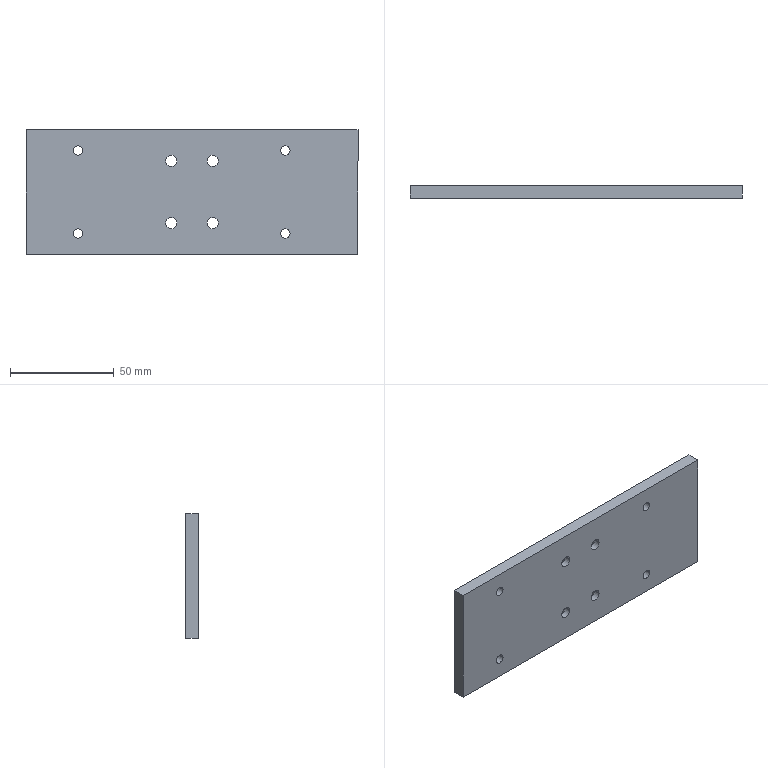Component | SolidWorks | CS021-A10-A007-1 | 1 solid | 30 faces | box 160 x 6 x 60 mm | volume 56270 mm3 | cylinder 16 | cone 8 | plane 6 | commonest cylinder face diameters 4.5 x8 5.5 x8 | material AL6061
build123d program:
from build123d import *

# Parameters (mm, degrees)
SKETCH1_W                                          = 160
SKETCH1_H                                          = 60
BOSS_EXTRUDE1_DEPTH                                = 3
HOLE_SIZE_ACCORDING_TO_SLOTTED_COUNTER_D           = 5.5
HOLE_SIZE_ACCORDING_TO_SLOTTED_COUNTER_CSINK_D     = 11.2
HOLE_SIZE_ACCORDING_TO_SLOTTED_COUNTER_CSINK_ANGLE = 90
F_4_5_4_5_DIAMETER_HOLE1_D                         = 4.5


with BuildPart() as part:
    # Sketch1 → Boss-Extrude1 (new, symmetric)
    with BuildSketch(Plane.XY):
        Rectangle(SKETCH1_W, SKETCH1_H)
    extrude(amount=BOSS_EXTRUDE1_DEPTH, both=True)

    # Hole Size _according to_ Slotted Counter (through all)
    with Locations(Plane.XY.offset(3)):
        with Locations((-10, 15), (10, 15), (10, -15), (-10, -15)):
            CounterSinkHole(HOLE_SIZE_ACCORDING_TO_SLOTTED_COUNTER_D / 2, HOLE_SIZE_ACCORDING_TO_SLOTTED_COUNTER_CSINK_D / 2, counter_sink_angle=HOLE_SIZE_ACCORDING_TO_SLOTTED_COUNTER_CSINK_ANGLE)

    # 4.5 _4.5_ Diameter Hole1 (through all)
    with Locations(Plane.XY.offset(3)):
        with Locations((-55.001, 20), (44.999, 20), (44.999, -20), (-55.001, -20)):
            Hole(F_4_5_4_5_DIAMETER_HOLE1_D / 2)


solid = part.part

# Placed as in the assembly
solid = solid.moved(Location((152.449, 155.317, 0), (-90, 0, 0)))
STEP:
#1=COLOUR_RGB('',0.7922,0.8196,0.9333);
#2=FILL_AREA_STYLE_COLOUR('',#1);
#3=FILL_AREA_STYLE('',(#2));
#4=SURFACE_STYLE_FILL_AREA(#3);
#5=SURFACE_SIDE_STYLE('',(#4));
#6=SURFACE_STYLE_USAGE(.BOTH.,#5);
#7=PRESENTATION_STYLE_ASSIGNMENT((#6));
#8=CARTESIAN_POINT('',(3.748,5.997,-0.7874));
#9=VERTEX_POINT('',#8);
#10=CARTESIAN_POINT('',(3.925,5.997,-0.7874));
#11=VERTEX_POINT('',#10);
#12=CARTESIAN_POINT('',(3.837,5.997,-0.7874));
#13=DIRECTION('',(-0.,1.,0.));
#14=DIRECTION('',(1.,0.,-0.));
#15=AXIS2_PLACEMENT_3D('',#12,#13,#14);
#16=CIRCLE('',#15,0.08858);
#17=EDGE_CURVE('',#9,#11,#16,.T.);
#18=ORIENTED_EDGE('',*,*,#17,.F.);
#19=CARTESIAN_POINT('',(3.748,6.233,-0.7874));
#20=VERTEX_POINT('',#19);
#21=CARTESIAN_POINT('',(3.748,6.233,-0.7874));
#22=DIRECTION('',(-0.,1.,0.));
#23=VECTOR('',#22,39.37);
#24=LINE('',#21,#23);
#25=EDGE_CURVE('',#9,#20,#24,.T.);
#26=ORIENTED_EDGE('',*,*,#25,.T.);
#27=CARTESIAN_POINT('',(3.925,6.233,-0.7874));
#28=VERTEX_POINT('',#27);
#29=CARTESIAN_POINT('',(3.837,6.233,-0.7874));
#30=DIRECTION('',(-0.,1.,0.));
#31=DIRECTION('',(1.,0.,-0.));
#32=AXIS2_PLACEMENT_3D('',#29,#30,#31);
#33=CIRCLE('',#32,0.08858);
#34=EDGE_CURVE('',#20,#28,#33,.T.);
#35=ORIENTED_EDGE('',*,*,#34,.T.);
#36=CARTESIAN_POINT('',(3.925,6.233,-0.7874));
#37=DIRECTION('',(-0.,1.,0.));
#38=VECTOR('',#37,39.37);
#39=LINE('',#36,#38);
#40=EDGE_CURVE('',#11,#28,#39,.T.);
#41=ORIENTED_EDGE('',*,*,#40,.F.);
#42=EDGE_LOOP('',(#18,#26,#35,#41));
#43=FACE_OUTER_BOUND('',#42,.T.);
#44=CARTESIAN_POINT('',(3.837,6.233,-0.7874));
#45=DIRECTION('',(-0.,1.,0.));
#46=DIRECTION('',(1.,0.,-0.));
#47=AXIS2_PLACEMENT_3D('',#44,#45,#46);
#48=CYLINDRICAL_SURFACE('',#47,0.08858);
#49=ADVANCED_FACE('',(#43),#48,.F.);
#50=CARTESIAN_POINT('',(7.685,5.997,-0.7874));
#51=VERTEX_POINT('',#50);
#52=CARTESIAN_POINT('',(7.862,5.997,-0.7874));
#53=VERTEX_POINT('',#52);
#54=CARTESIAN_POINT('',(7.774,5.997,-0.7874));
#55=DIRECTION('',(-0.,1.,0.));
#56=DIRECTION('',(1.,0.,-0.));
#57=AXIS2_PLACEMENT_3D('',#54,#55,#56);
#58=CIRCLE('',#57,0.08858);
#59=EDGE_CURVE('',#51,#53,#58,.T.);
#60=ORIENTED_EDGE('',*,*,#59,.F.);
#61=CARTESIAN_POINT('',(7.685,6.233,-0.7874));
#62=VERTEX_POINT('',#61);
#63=CARTESIAN_POINT('',(7.685,6.233,-0.7874));
#64=DIRECTION('',(-0.,1.,0.));
#65=VECTOR('',#64,39.37);
#66=LINE('',#63,#65);
#67=EDGE_CURVE('',#51,#62,#66,.T.);
#68=ORIENTED_EDGE('',*,*,#67,.T.);
#69=CARTESIAN_POINT('',(7.862,6.233,-0.7874));
#70=VERTEX_POINT('',#69);
#71=CARTESIAN_POINT('',(7.774,6.233,-0.7874));
#72=DIRECTION('',(-0.,1.,0.));
#73=DIRECTION('',(1.,0.,-0.));
#74=AXIS2_PLACEMENT_3D('',#71,#72,#73);
#75=CIRCLE('',#74,0.08858);
#76=EDGE_CURVE('',#62,#70,#75,.T.);
#77=ORIENTED_EDGE('',*,*,#76,.T.);
#78=CARTESIAN_POINT('',(7.862,6.233,-0.7874));
#79=DIRECTION('',(-0.,1.,0.));
#80=VECTOR('',#79,39.37);
#81=LINE('',#78,#80);
#82=EDGE_CURVE('',#53,#70,#81,.T.);
#83=ORIENTED_EDGE('',*,*,#82,.F.);
#84=EDGE_LOOP('',(#60,#68,#77,#83));
#85=FACE_OUTER_BOUND('',#84,.T.);
#86=CARTESIAN_POINT('',(7.774,6.233,-0.7874));
#87=DIRECTION('',(-0.,1.,0.));
#88=DIRECTION('',(1.,0.,-0.));
#89=AXIS2_PLACEMENT_3D('',#86,#87,#88);
#90=CYLINDRICAL_SURFACE('',#89,0.08858);
#91=ADVANCED_FACE('',(#85),#90,.F.);
#92=CARTESIAN_POINT('',(7.685,5.997,0.7874));
#93=VERTEX_POINT('',#92);
#94=CARTESIAN_POINT('',(7.862,5.997,0.7874));
#95=VERTEX_POINT('',#94);
#96=CARTESIAN_POINT('',(7.774,5.997,0.7874));
#97=DIRECTION('',(-0.,1.,0.));
#98=DIRECTION('',(1.,0.,-0.));
#99=AXIS2_PLACEMENT_3D('',#96,#97,#98);
#100=CIRCLE('',#99,0.08858);
#101=EDGE_CURVE('',#93,#95,#100,.T.);
#102=ORIENTED_EDGE('',*,*,#101,.F.);
#103=CARTESIAN_POINT('',(7.685,6.233,0.7874));
#104=VERTEX_POINT('',#103);
#105=CARTESIAN_POINT('',(7.685,6.233,0.7874));
#106=DIRECTION('',(-0.,1.,0.));
#107=VECTOR('',#106,39.37);
#108=LINE('',#105,#107);
#109=EDGE_CURVE('',#93,#104,#108,.T.);
#110=ORIENTED_EDGE('',*,*,#109,.T.);
#111=CARTESIAN_POINT('',(7.862,6.233,0.7874));
#112=VERTEX_POINT('',#111);
#113=CARTESIAN_POINT('',(7.774,6.233,0.7874));
#114=DIRECTION('',(-0.,1.,0.));
#115=DIRECTION('',(1.,0.,-0.));
#116=AXIS2_PLACEMENT_3D('',#113,#114,#115);
#117=CIRCLE('',#116,0.08858);
#118=EDGE_CURVE('',#104,#112,#117,.T.);
#119=ORIENTED_EDGE('',*,*,#118,.T.);
#120=CARTESIAN_POINT('',(7.862,6.233,0.7874));
#121=DIRECTION('',(-0.,1.,0.));
#122=VECTOR('',#121,39.37);
#123=LINE('',#120,#122);
#124=EDGE_CURVE('',#95,#112,#123,.T.);
#125=ORIENTED_EDGE('',*,*,#124,.F.);
#126=EDGE_LOOP('',(#102,#110,#119,#125));
#127=FACE_OUTER_BOUND('',#126,.T.);
#128=CARTESIAN_POINT('',(7.774,6.233,0.7874));
#129=DIRECTION('',(-0.,1.,0.));
#130=DIRECTION('',(1.,0.,-0.));
#131=AXIS2_PLACEMENT_3D('',#128,#129,#130);
#132=CYLINDRICAL_SURFACE('',#131,0.08858);
#133=ADVANCED_FACE('',(#127),#132,.F.);
#134=CARTESIAN_POINT('',(3.748,5.997,0.7874));
#135=VERTEX_POINT('',#134);
#136=CARTESIAN_POINT('',(3.925,5.997,0.7874));
#137=VERTEX_POINT('',#136);
#138=CARTESIAN_POINT('',(3.837,5.997,0.7874));
#139=DIRECTION('',(-0.,1.,0.));
#140=DIRECTION('',(1.,0.,-0.));
#141=AXIS2_PLACEMENT_3D('',#138,#139,#140);
#142=CIRCLE('',#141,0.08858);
#143=EDGE_CURVE('',#135,#137,#142,.T.);
#144=ORIENTED_EDGE('',*,*,#143,.F.);
#145=CARTESIAN_POINT('',(3.748,6.233,0.7874));
#146=VERTEX_POINT('',#145);
#147=CARTESIAN_POINT('',(3.748,6.233,0.7874));
#148=DIRECTION('',(-0.,1.,0.));
#149=VECTOR('',#148,39.37);
#150=LINE('',#147,#149);
#151=EDGE_CURVE('',#135,#146,#150,.T.);
#152=ORIENTED_EDGE('',*,*,#151,.T.);
#153=CARTESIAN_POINT('',(3.925,6.233,0.7874));
#154=VERTEX_POINT('',#153);
#155=CARTESIAN_POINT('',(3.837,6.233,0.7874));
#156=DIRECTION('',(-0.,1.,0.));
#157=DIRECTION('',(1.,0.,-0.));
#158=AXIS2_PLACEMENT_3D('',#155,#156,#157);
#159=CIRCLE('',#158,0.08858);
#160=EDGE_CURVE('',#146,#154,#159,.T.);
#161=ORIENTED_EDGE('',*,*,#160,.T.);
#162=CARTESIAN_POINT('',(3.925,6.233,0.7874));
#163=DIRECTION('',(-0.,1.,0.));
#164=VECTOR('',#163,39.37);
#165=LINE('',#162,#164);
#166=EDGE_CURVE('',#137,#154,#165,.T.);
#167=ORIENTED_EDGE('',*,*,#166,.F.);
#168=EDGE_LOOP('',(#144,#152,#161,#167));
#169=FACE_OUTER_BOUND('',#168,.T.);
#170=CARTESIAN_POINT('',(3.837,6.233,0.7874));
#171=DIRECTION('',(-0.,1.,0.));
#172=DIRECTION('',(1.,0.,-0.));
#173=AXIS2_PLACEMENT_3D('',#170,#171,#172);
#174=CYLINDRICAL_SURFACE('',#173,0.08858);
#175=ADVANCED_FACE('',(#169),#174,.F.);
#176=CARTESIAN_POINT('',(5.5,6.121,-0.5906));
#177=VERTEX_POINT('',#176);
#178=CARTESIAN_POINT('',(5.716,6.121,-0.5906));
#179=VERTEX_POINT('',#178);
#180=CARTESIAN_POINT('',(5.608,6.121,-0.5906));
#181=DIRECTION('',(-0.,1.,0.));
#182=DIRECTION('',(1.,0.,-0.));
#183=AXIS2_PLACEMENT_3D('',#180,#181,#182);
#184=CIRCLE('',#183,0.1083);
#185=EDGE_CURVE('',#177,#179,#184,.T.);
#186=ORIENTED_EDGE('',*,*,#185,.F.);
#187=CARTESIAN_POINT('',(5.388,6.233,-0.5906));
#188=VERTEX_POINT('',#187);
#189=CARTESIAN_POINT('',(5.388,6.233,-0.5906));
#190=DIRECTION('',(-0.7071,0.7071,0.));
#191=VECTOR('',#190,39.37);
#192=LINE('',#189,#191);
#193=EDGE_CURVE('',#177,#188,#192,.T.);
#194=ORIENTED_EDGE('',*,*,#193,.T.);
#195=CARTESIAN_POINT('',(5.829,6.233,-0.5906));
#196=VERTEX_POINT('',#195);
#197=CARTESIAN_POINT('',(5.608,6.233,-0.5906));
#198=DIRECTION('',(-0.,1.,0.));
#199=DIRECTION('',(1.,0.,-0.));
#200=AXIS2_PLACEMENT_3D('',#197,#198,#199);
#201=CIRCLE('',#200,0.2205);
#202=EDGE_CURVE('',#188,#196,#201,.T.);
#203=ORIENTED_EDGE('',*,*,#202,.T.);
#204=CARTESIAN_POINT('',(5.829,6.233,-0.5906));
#205=DIRECTION('',(0.7071,0.7071,-0.));
#206=VECTOR('',#205,39.37);
#207=LINE('',#204,#206);
#208=EDGE_CURVE('',#179,#196,#207,.T.);
#209=ORIENTED_EDGE('',*,*,#208,.F.);
#210=EDGE_LOOP('',(#186,#194,#203,#209));
#211=FACE_OUTER_BOUND('',#210,.T.);
#212=CARTESIAN_POINT('',(5.608,6.233,-0.5906));
#213=DIRECTION('',(-0.,1.,0.));
#214=DIRECTION('',(1.,0.,-0.));
#215=AXIS2_PLACEMENT_3D('',#212,#213,#214);
#216=CONICAL_SURFACE('',#215,0.2205,0.7854);
#217=ADVANCED_FACE('',(#211),#216,.F.);
#218=CARTESIAN_POINT('',(5.5,5.997,-0.5906));
#219=VERTEX_POINT('',#218);
#220=CARTESIAN_POINT('',(5.716,5.997,-0.5906));
#221=VERTEX_POINT('',#220);
#222=CARTESIAN_POINT('',(5.608,5.997,-0.5906));
#223=DIRECTION('',(-0.,1.,0.));
#224=DIRECTION('',(1.,0.,-0.));
#225=AXIS2_PLACEMENT_3D('',#222,#223,#224);
#226=CIRCLE('',#225,0.1083);
#227=EDGE_CURVE('',#219,#221,#226,.T.);
#228=ORIENTED_EDGE('',*,*,#227,.F.);
#229=CARTESIAN_POINT('',(5.5,6.233,-0.5906));
#230=DIRECTION('',(-0.,1.,0.));
#231=VECTOR('',#230,39.37);
#232=LINE('',#229,#231);
#233=EDGE_CURVE('',#219,#177,#232,.T.);
#234=ORIENTED_EDGE('',*,*,#233,.T.);
#235=ORIENTED_EDGE('',*,*,#185,.T.);
#236=CARTESIAN_POINT('',(5.716,6.233,-0.5906));
#237=DIRECTION('',(-0.,1.,0.));
#238=VECTOR('',#237,39.37);
#239=LINE('',#236,#238);
#240=EDGE_CURVE('',#221,#179,#239,.T.);
#241=ORIENTED_EDGE('',*,*,#240,.F.);
#242=EDGE_LOOP('',(#228,#234,#235,#241));
#243=FACE_OUTER_BOUND('',#242,.T.);
#244=CARTESIAN_POINT('',(5.608,6.233,-0.5906));
#245=DIRECTION('',(-0.,1.,0.));
#246=DIRECTION('',(1.,0.,-0.));
#247=AXIS2_PLACEMENT_3D('',#244,#245,#246);
#248=CYLINDRICAL_SURFACE('',#247,0.1083);
#249=ADVANCED_FACE('',(#243),#248,.F.);
#250=CARTESIAN_POINT('',(6.287,6.121,-0.5906));
#251=VERTEX_POINT('',#250);
#252=CARTESIAN_POINT('',(6.504,6.121,-0.5906));
#253=VERTEX_POINT('',#252);
#254=CARTESIAN_POINT('',(6.396,6.121,-0.5906));
#255=DIRECTION('',(-0.,1.,0.));
#256=DIRECTION('',(1.,0.,-0.));
#257=AXIS2_PLACEMENT_3D('',#254,#255,#256);
#258=CIRCLE('',#257,0.1083);
#259=EDGE_CURVE('',#251,#253,#258,.T.);
#260=ORIENTED_EDGE('',*,*,#259,.F.);
#261=CARTESIAN_POINT('',(6.175,6.233,-0.5906));
#262=VERTEX_POINT('',#261);
#263=CARTESIAN_POINT('',(6.175,6.233,-0.5906));
#264=DIRECTION('',(-0.7071,0.7071,0.));
#265=VECTOR('',#264,39.37);
#266=LINE('',#263,#265);
#267=EDGE_CURVE('',#251,#262,#266,.T.);
#268=ORIENTED_EDGE('',*,*,#267,.T.);
#269=CARTESIAN_POINT('',(6.616,6.233,-0.5906));
#270=VERTEX_POINT('',#269);
#271=CARTESIAN_POINT('',(6.396,6.233,-0.5906));
#272=DIRECTION('',(-0.,1.,0.));
#273=DIRECTION('',(1.,0.,-0.));
#274=AXIS2_PLACEMENT_3D('',#271,#272,#273);
#275=CIRCLE('',#274,0.2205);
#276=EDGE_CURVE('',#262,#270,#275,.T.);
#277=ORIENTED_EDGE('',*,*,#276,.T.);
#278=CARTESIAN_POINT('',(6.616,6.233,-0.5906));
#279=DIRECTION('',(0.7071,0.7071,-0.));
#280=VECTOR('',#279,39.37);
#281=LINE('',#278,#280);
#282=EDGE_CURVE('',#253,#270,#281,.T.);
#283=ORIENTED_EDGE('',*,*,#282,.F.);
#284=EDGE_LOOP('',(#260,#268,#277,#283));
#285=FACE_OUTER_BOUND('',#284,.T.);
#286=CARTESIAN_POINT('',(6.396,6.233,-0.5906));
#287=DIRECTION('',(-0.,1.,0.));
#288=DIRECTION('',(1.,0.,-0.));
#289=AXIS2_PLACEMENT_3D('',#286,#287,#288);
#290=CONICAL_SURFACE('',#289,0.2205,0.7854);
#291=ADVANCED_FACE('',(#285),#290,.F.);
#292=CARTESIAN_POINT('',(6.287,5.997,-0.5906));
#293=VERTEX_POINT('',#292);
#294=CARTESIAN_POINT('',(6.504,5.997,-0.5906));
#295=VERTEX_POINT('',#294);
#296=CARTESIAN_POINT('',(6.396,5.997,-0.5906));
#297=DIRECTION('',(-0.,1.,0.));
#298=DIRECTION('',(1.,0.,-0.));
#299=AXIS2_PLACEMENT_3D('',#296,#297,#298);
#300=CIRCLE('',#299,0.1083);
#301=EDGE_CURVE('',#293,#295,#300,.T.);
#302=ORIENTED_EDGE('',*,*,#301,.F.);
#303=CARTESIAN_POINT('',(6.287,6.233,-0.5906));
#304=DIRECTION('',(-0.,1.,0.));
#305=VECTOR('',#304,39.37);
#306=LINE('',#303,#305);
#307=EDGE_CURVE('',#293,#251,#306,.T.);
#308=ORIENTED_EDGE('',*,*,#307,.T.);
#309=ORIENTED_EDGE('',*,*,#259,.T.);
#310=CARTESIAN_POINT('',(6.504,6.233,-0.5906));
#311=DIRECTION('',(-0.,1.,0.));
#312=VECTOR('',#311,39.37);
#313=LINE('',#310,#312);
#314=EDGE_CURVE('',#295,#253,#313,.T.);
#315=ORIENTED_EDGE('',*,*,#314,.F.);
#316=EDGE_LOOP('',(#302,#308,#309,#315));
#317=FACE_OUTER_BOUND('',#316,.T.);
#318=CARTESIAN_POINT('',(6.396,6.233,-0.5906));
#319=DIRECTION('',(-0.,1.,0.));
#320=DIRECTION('',(1.,0.,-0.));
#321=AXIS2_PLACEMENT_3D('',#318,#319,#320);
#322=CYLINDRICAL_SURFACE('',#321,0.1083);
#323=ADVANCED_FACE('',(#317),#322,.F.);
#324=CARTESIAN_POINT('',(6.287,6.121,0.5906));
#325=VERTEX_POINT('',#324);
#326=CARTESIAN_POINT('',(6.504,6.121,0.5906));
#327=VERTEX_POINT('',#326);
#328=CARTESIAN_POINT('',(6.396,6.121,0.5906));
#329=DIRECTION('',(-0.,1.,0.));
#330=DIRECTION('',(1.,0.,-0.));
#331=AXIS2_PLACEMENT_3D('',#328,#329,#330);
#332=CIRCLE('',#331,0.1083);
#333=EDGE_CURVE('',#325,#327,#332,.T.);
#334=ORIENTED_EDGE('',*,*,#333,.F.);
#335=CARTESIAN_POINT('',(6.175,6.233,0.5906));
#336=VERTEX_POINT('',#335);
#337=CARTESIAN_POINT('',(6.175,6.233,0.5906));
#338=DIRECTION('',(-0.7071,0.7071,0.));
#339=VECTOR('',#338,39.37);
#340=LINE('',#337,#339);
#341=EDGE_CURVE('',#325,#336,#340,.T.);
#342=ORIENTED_EDGE('',*,*,#341,.T.);
#343=CARTESIAN_POINT('',(6.616,6.233,0.5906));
#344=VERTEX_POINT('',#343);
#345=CARTESIAN_POINT('',(6.396,6.233,0.5906));
#346=DIRECTION('',(-0.,1.,0.));
#347=DIRECTION('',(1.,0.,-0.));
#348=AXIS2_PLACEMENT_3D('',#345,#346,#347);
#349=CIRCLE('',#348,0.2205);
#350=EDGE_CURVE('',#336,#344,#349,.T.);
#351=ORIENTED_EDGE('',*,*,#350,.T.);
#352=CARTESIAN_POINT('',(6.616,6.233,0.5906));
#353=DIRECTION('',(0.7071,0.7071,-0.));
#354=VECTOR('',#353,39.37);
#355=LINE('',#352,#354);
#356=EDGE_CURVE('',#327,#344,#355,.T.);
#357=ORIENTED_EDGE('',*,*,#356,.F.);
#358=EDGE_LOOP('',(#334,#342,#351,#357));
#359=FACE_OUTER_BOUND('',#358,.T.);
#360=CARTESIAN_POINT('',(6.396,6.233,0.5906));
#361=DIRECTION('',(-0.,1.,0.));
#362=DIRECTION('',(1.,0.,-0.));
#363=AXIS2_PLACEMENT_3D('',#360,#361,#362);
#364=CONICAL_SURFACE('',#363,0.2205,0.7854);
#365=ADVANCED_FACE('',(#359),#364,.F.);
#366=CARTESIAN_POINT('',(6.287,5.997,0.5906));
#367=VERTEX_POINT('',#366);
#368=CARTESIAN_POINT('',(6.504,5.997,0.5906));
#369=VERTEX_POINT('',#368);
#370=CARTESIAN_POINT('',(6.396,5.997,0.5906));
#371=DIRECTION('',(-0.,1.,0.));
#372=DIRECTION('',(1.,0.,-0.));
#373=AXIS2_PLACEMENT_3D('',#370,#371,#372);
#374=CIRCLE('',#373,0.1083);
#375=EDGE_CURVE('',#367,#369,#374,.T.);
#376=ORIENTED_EDGE('',*,*,#375,.F.);
#377=CARTESIAN_POINT('',(6.287,6.233,0.5906));
#378=DIRECTION('',(-0.,1.,0.));
#379=VECTOR('',#378,39.37);
#380=LINE('',#377,#379);
#381=EDGE_CURVE('',#367,#325,#380,.T.);
#382=ORIENTED_EDGE('',*,*,#381,.T.);
#383=ORIENTED_EDGE('',*,*,#333,.T.);
#384=CARTESIAN_POINT('',(6.504,6.233,0.5906));
#385=DIRECTION('',(-0.,1.,0.));
#386=VECTOR('',#385,39.37);
#387=LINE('',#384,#386);
#388=EDGE_CURVE('',#369,#327,#387,.T.);
#389=ORIENTED_EDGE('',*,*,#388,.F.);
#390=EDGE_LOOP('',(#376,#382,#383,#389));
#391=FACE_OUTER_BOUND('',#390,.T.);
#392=CARTESIAN_POINT('',(6.396,6.233,0.5906));
#393=DIRECTION('',(-0.,1.,0.));
#394=DIRECTION('',(1.,0.,-0.));
#395=AXIS2_PLACEMENT_3D('',#392,#393,#394);
#396=CYLINDRICAL_SURFACE('',#395,0.1083);
#397=ADVANCED_FACE('',(#391),#396,.F.);
#398=CARTESIAN_POINT('',(5.5,6.121,0.5906));
#399=VERTEX_POINT('',#398);
#400=CARTESIAN_POINT('',(5.716,6.121,0.5906));
#401=VERTEX_POINT('',#400);
#402=CARTESIAN_POINT('',(5.608,6.121,0.5906));
#403=DIRECTION('',(-0.,1.,0.));
#404=DIRECTION('',(1.,0.,-0.));
#405=AXIS2_PLACEMENT_3D('',#402,#403,#404);
#406=CIRCLE('',#405,0.1083);
#407=EDGE_CURVE('',#399,#401,#406,.T.);
#408=ORIENTED_EDGE('',*,*,#407,.F.);
#409=CARTESIAN_POINT('',(5.388,6.233,0.5906));
#410=VERTEX_POINT('',#409);
#411=CARTESIAN_POINT('',(5.388,6.233,0.5906));
#412=DIRECTION('',(-0.7071,0.7071,0.));
#413=VECTOR('',#412,39.37);
#414=LINE('',#411,#413);
#415=EDGE_CURVE('',#399,#410,#414,.T.);
#416=ORIENTED_EDGE('',*,*,#415,.T.);
#417=CARTESIAN_POINT('',(5.829,6.233,0.5906));
#418=VERTEX_POINT('',#417);
#419=CARTESIAN_POINT('',(5.608,6.233,0.5906));
#420=DIRECTION('',(-0.,1.,0.));
#421=DIRECTION('',(1.,0.,-0.));
#422=AXIS2_PLACEMENT_3D('',#419,#420,#421);
#423=CIRCLE('',#422,0.2205);
#424=EDGE_CURVE('',#410,#418,#423,.T.);
#425=ORIENTED_EDGE('',*,*,#424,.T.);
#426=CARTESIAN_POINT('',(5.829,6.233,0.5906));
#427=DIRECTION('',(0.7071,0.7071,-0.));
#428=VECTOR('',#427,39.37);
#429=LINE('',#426,#428);
#430=EDGE_CURVE('',#401,#418,#429,.T.);
#431=ORIENTED_EDGE('',*,*,#430,.F.);
#432=EDGE_LOOP('',(#408,#416,#425,#431));
#433=FACE_OUTER_BOUND('',#432,.T.);
#434=CARTESIAN_POINT('',(5.608,6.233,0.5906));
#435=DIRECTION('',(-0.,1.,0.));
#436=DIRECTION('',(1.,0.,-0.));
#437=AXIS2_PLACEMENT_3D('',#434,#435,#436);
#438=CONICAL_SURFACE('',#437,0.2205,0.7854);
#439=ADVANCED_FACE('',(#433),#438,.F.);
#440=CARTESIAN_POINT('',(5.5,5.997,0.5906));
#441=VERTEX_POINT('',#440);
#442=CARTESIAN_POINT('',(5.716,5.997,0.5906));
#443=VERTEX_POINT('',#442);
#444=CARTESIAN_POINT('',(5.608,5.997,0.5906));
#445=DIRECTION('',(-0.,1.,0.));
#446=DIRECTION('',(1.,0.,-0.));
#447=AXIS2_PLACEMENT_3D('',#444,#445,#446);
#448=CIRCLE('',#447,0.1083);
#449=EDGE_CURVE('',#441,#443,#448,.T.);
#450=ORIENTED_EDGE('',*,*,#449,.F.);
#451=CARTESIAN_POINT('',(5.5,6.233,0.5906));
#452=DIRECTION('',(-0.,1.,0.));
#453=VECTOR('',#452,39.37);
#454=LINE('',#451,#453);
#455=EDGE_CURVE('',#441,#399,#454,.T.);
#456=ORIENTED_EDGE('',*,*,#455,.T.);
#457=ORIENTED_EDGE('',*,*,#407,.T.);
#458=CARTESIAN_POINT('',(5.716,6.233,0.5906));
#459=DIRECTION('',(-0.,1.,0.));
#460=VECTOR('',#459,39.37);
#461=LINE('',#458,#460);
#462=EDGE_CURVE('',#443,#401,#461,.T.);
#463=ORIENTED_EDGE('',*,*,#462,.F.);
#464=EDGE_LOOP('',(#450,#456,#457,#463));
#465=FACE_OUTER_BOUND('',#464,.T.);
#466=CARTESIAN_POINT('',(5.608,6.233,0.5906));
#467=DIRECTION('',(-0.,1.,0.));
#468=DIRECTION('',(1.,0.,-0.));
#469=AXIS2_PLACEMENT_3D('',#466,#467,#468);
#470=CYLINDRICAL_SURFACE('',#469,0.1083);
#471=ADVANCED_FACE('',(#465),#470,.F.);
#472=CARTESIAN_POINT('',(3.837,6.233,-0.7874));
#473=DIRECTION('',(-0.,1.,0.));
#474=DIRECTION('',(1.,0.,-0.));
#475=AXIS2_PLACEMENT_3D('',#472,#473,#474);
#476=CIRCLE('',#475,0.08858);
#477=EDGE_CURVE('',#28,#20,#476,.T.);
#478=ORIENTED_EDGE('',*,*,#477,.F.);
#479=ORIENTED_EDGE('',*,*,#34,.F.);
#480=EDGE_LOOP('',(#478,#479));
#481=FACE_BOUND('',#480,.T.);
#482=CARTESIAN_POINT('',(7.774,6.233,-0.7874));
#483=DIRECTION('',(-0.,1.,0.));
#484=DIRECTION('',(1.,0.,-0.));
#485=AXIS2_PLACEMENT_3D('',#482,#483,#484);
#486=CIRCLE('',#485,0.08858);
#487=EDGE_CURVE('',#70,#62,#486,.T.);
#488=ORIENTED_EDGE('',*,*,#487,.F.);
#489=ORIENTED_EDGE('',*,*,#76,.F.);
#490=EDGE_LOOP('',(#488,#489));
#491=FACE_BOUND('',#490,.T.);
#492=CARTESIAN_POINT('',(7.774,6.233,0.7874));
#493=DIRECTION('',(-0.,1.,0.));
#494=DIRECTION('',(1.,0.,-0.));
#495=AXIS2_PLACEMENT_3D('',#492,#493,#494);
#496=CIRCLE('',#495,0.08858);
#497=EDGE_CURVE('',#112,#104,#496,.T.);
#498=ORIENTED_EDGE('',*,*,#497,.F.);
#499=ORIENTED_EDGE('',*,*,#118,.F.);
#500=EDGE_LOOP('',(#498,#499));
#501=FACE_BOUND('',#500,.T.);
#502=CARTESIAN_POINT('',(9.152,6.233,1.181));
#503=VERTEX_POINT('',#502);
#504=CARTESIAN_POINT('',(9.152,6.233,-1.181));
#505=VERTEX_POINT('',#504);
#506=CARTESIAN_POINT('',(9.152,6.233,1.181));
#507=DIRECTION('',(-0.,0.,-1.));
#508=VECTOR('',#507,39.37);
#509=LINE('',#506,#508);
#510=EDGE_CURVE('',#503,#505,#509,.T.);
#511=ORIENTED_EDGE('',*,*,#510,.T.);
#512=CARTESIAN_POINT('',(2.852,6.233,-1.181));
#513=VERTEX_POINT('',#512);
#514=CARTESIAN_POINT('',(2.852,6.233,-1.181));
#515=DIRECTION('',(-1.,-0.,0.));
#516=VECTOR('',#515,39.37);
#517=LINE('',#514,#516);
#518=EDGE_CURVE('',#505,#513,#517,.T.);
#519=ORIENTED_EDGE('',*,*,#518,.T.);
#520=CARTESIAN_POINT('',(2.852,6.233,1.181));
#521=VERTEX_POINT('',#520);
#522=CARTESIAN_POINT('',(2.852,6.233,1.181));
#523=DIRECTION('',(0.,-0.,1.));
#524=VECTOR('',#523,39.37);
#525=LINE('',#522,#524);
#526=EDGE_CURVE('',#513,#521,#525,.T.);
#527=ORIENTED_EDGE('',*,*,#526,.T.);
#528=CARTESIAN_POINT('',(2.852,6.233,1.181));
#529=DIRECTION('',(1.,0.,-0.));
#530=VECTOR('',#529,39.37);
#531=LINE('',#528,#530);
#532=EDGE_CURVE('',#521,#503,#531,.T.);
#533=ORIENTED_EDGE('',*,*,#532,.T.);
#534=EDGE_LOOP('',(#511,#519,#527,#533));
#535=FACE_OUTER_BOUND('',#534,.T.);
#536=CARTESIAN_POINT('',(5.608,6.233,0.5906));
#537=DIRECTION('',(-0.,1.,0.));
#538=DIRECTION('',(1.,0.,-0.));
#539=AXIS2_PLACEMENT_3D('',#536,#537,#538);
#540=CIRCLE('',#539,0.2205);
#541=EDGE_CURVE('',#418,#410,#540,.T.);
#542=ORIENTED_EDGE('',*,*,#541,.F.);
#543=ORIENTED_EDGE('',*,*,#424,.F.);
#544=EDGE_LOOP('',(#542,#543));
#545=FACE_BOUND('',#544,.T.);
#546=CARTESIAN_POINT('',(6.396,6.233,0.5906));
#547=DIRECTION('',(-0.,1.,0.));
#548=DIRECTION('',(1.,0.,-0.));
#549=AXIS2_PLACEMENT_3D('',#546,#547,#548);
#550=CIRCLE('',#549,0.2205);
#551=EDGE_CURVE('',#344,#336,#550,.T.);
#552=ORIENTED_EDGE('',*,*,#551,.F.);
#553=ORIENTED_EDGE('',*,*,#350,.F.);
#554=EDGE_LOOP('',(#552,#553));
#555=FACE_BOUND('',#554,.T.);
#556=CARTESIAN_POINT('',(6.396,6.233,-0.5906));
#557=DIRECTION('',(-0.,1.,0.));
#558=DIRECTION('',(1.,0.,-0.));
#559=AXIS2_PLACEMENT_3D('',#556,#557,#558);
#560=CIRCLE('',#559,0.2205);
#561=EDGE_CURVE('',#270,#262,#560,.T.);
#562=ORIENTED_EDGE('',*,*,#561,.F.);
#563=ORIENTED_EDGE('',*,*,#276,.F.);
#564=EDGE_LOOP('',(#562,#563));
#565=FACE_BOUND('',#564,.T.);
#566=CARTESIAN_POINT('',(5.608,6.233,-0.5906));
#567=DIRECTION('',(-0.,1.,0.));
#568=DIRECTION('',(1.,0.,-0.));
#569=AXIS2_PLACEMENT_3D('',#566,#567,#568);
#570=CIRCLE('',#569,0.2205);
#571=EDGE_CURVE('',#196,#188,#570,.T.);
#572=ORIENTED_EDGE('',*,*,#571,.F.);
#573=ORIENTED_EDGE('',*,*,#202,.F.);
#574=EDGE_LOOP('',(#572,#573));
#575=FACE_BOUND('',#574,.T.);
#576=CARTESIAN_POINT('',(3.837,6.233,0.7874));
#577=DIRECTION('',(-0.,1.,0.));
#578=DIRECTION('',(1.,0.,-0.));
#579=AXIS2_PLACEMENT_3D('',#576,#577,#578);
#580=CIRCLE('',#579,0.08858);
#581=EDGE_CURVE('',#154,#146,#580,.T.);
#582=ORIENTED_EDGE('',*,*,#581,.F.);
#583=ORIENTED_EDGE('',*,*,#160,.F.);
#584=EDGE_LOOP('',(#582,#583));
#585=FACE_BOUND('',#584,.T.);
#586=CARTESIAN_POINT('',(6.002,6.233,0.));
#587=DIRECTION('',(0.,-1.,-0.));
#588=DIRECTION('',(-1.,-0.,0.));
#589=AXIS2_PLACEMENT_3D('',#586,#587,#588);
#590=PLANE('',#589);
#591=ADVANCED_FACE('',(#481,#491,#501,#535,#545,#555,#565,#575,#585),#590,.F.);
#592=CARTESIAN_POINT('',(9.152,5.997,1.181));
#593=VERTEX_POINT('',#592);
#594=CARTESIAN_POINT('',(9.152,5.997,-1.181));
#595=VERTEX_POINT('',#594);
#596=CARTESIAN_POINT('',(9.152,5.997,1.181));
#597=DIRECTION('',(-0.,0.,-1.));
#598=VECTOR('',#597,39.37);
#599=LINE('',#596,#598);
#600=EDGE_CURVE('',#593,#595,#599,.T.);
#601=ORIENTED_EDGE('',*,*,#600,.T.);
#602=CARTESIAN_POINT('',(9.152,6.233,-1.181));
#603=DIRECTION('',(0.,-1.,-0.));
#604=VECTOR('',#603,39.37);
#605=LINE('',#602,#604);
#606=EDGE_CURVE('',#505,#595,#605,.T.);
#607=ORIENTED_EDGE('',*,*,#606,.F.);
#608=ORIENTED_EDGE('',*,*,#510,.F.);
#609=CARTESIAN_POINT('',(9.152,6.233,1.181));
#610=DIRECTION('',(0.,-1.,-0.));
#611=VECTOR('',#610,39.37);
#612=LINE('',#609,#611);
#613=EDGE_CURVE('',#503,#593,#612,.T.);
#614=ORIENTED_EDGE('',*,*,#613,.T.);
#615=EDGE_LOOP('',(#601,#607,#608,#614));
#616=FACE_OUTER_BOUND('',#615,.T.);
#617=CARTESIAN_POINT('',(9.152,6.233,1.181));
#618=DIRECTION('',(-1.,-0.,0.));
#619=DIRECTION('',(-0.,1.,0.));
#620=AXIS2_PLACEMENT_3D('',#617,#618,#619);
#621=PLANE('',#620);
#622=ADVANCED_FACE('',(#616),#621,.F.);
#623=CARTESIAN_POINT('',(2.852,5.997,-1.181));
#624=VERTEX_POINT('',#623);
#625=CARTESIAN_POINT('',(2.852,5.997,-1.181));
#626=DIRECTION('',(-1.,-0.,0.));
#627=VECTOR('',#626,39.37);
#628=LINE('',#625,#627);
#629=EDGE_CURVE('',#595,#624,#628,.T.);
#630=ORIENTED_EDGE('',*,*,#629,.T.);
#631=CARTESIAN_POINT('',(2.852,6.233,-1.181));
#632=DIRECTION('',(0.,-1.,-0.));
#633=VECTOR('',#632,39.37);
#634=LINE('',#631,#633);
#635=EDGE_CURVE('',#513,#624,#634,.T.);
#636=ORIENTED_EDGE('',*,*,#635,.F.);
#637=ORIENTED_EDGE('',*,*,#518,.F.);
#638=ORIENTED_EDGE('',*,*,#606,.T.);
#639=EDGE_LOOP('',(#630,#636,#637,#638));
#640=FACE_OUTER_BOUND('',#639,.T.);
#641=CARTESIAN_POINT('',(2.852,6.233,-1.181));
#642=DIRECTION('',(0.,-0.,1.));
#643=DIRECTION('',(0.,-1.,-0.));
#644=AXIS2_PLACEMENT_3D('',#641,#642,#643);
#645=PLANE('',#644);
#646=ADVANCED_FACE('',(#640),#645,.F.);
#647=CARTESIAN_POINT('',(2.852,5.997,1.181));
#648=VERTEX_POINT('',#647);
#649=CARTESIAN_POINT('',(2.852,5.997,1.181));
#650=DIRECTION('',(0.,-0.,1.));
#651=VECTOR('',#650,39.37);
#652=LINE('',#649,#651);
#653=EDGE_CURVE('',#624,#648,#652,.T.);
#654=ORIENTED_EDGE('',*,*,#653,.T.);
#655=CARTESIAN_POINT('',(2.852,6.233,1.181));
#656=DIRECTION('',(0.,-1.,-0.));
#657=VECTOR('',#656,39.37);
#658=LINE('',#655,#657);
#659=EDGE_CURVE('',#521,#648,#658,.T.);
#660=ORIENTED_EDGE('',*,*,#659,.F.);
#661=ORIENTED_EDGE('',*,*,#526,.F.);
#662=ORIENTED_EDGE('',*,*,#635,.T.);
#663=EDGE_LOOP('',(#654,#660,#661,#662));
#664=FACE_OUTER_BOUND('',#663,.T.);
#665=CARTESIAN_POINT('',(2.852,6.233,1.181));
#666=DIRECTION('',(1.,0.,-0.));
#667=DIRECTION('',(0.,-1.,-0.));
#668=AXIS2_PLACEMENT_3D('',#665,#666,#667);
#669=PLANE('',#668);
#670=ADVANCED_FACE('',(#664),#669,.F.);
#671=CARTESIAN_POINT('',(2.852,5.997,1.181));
#672=DIRECTION('',(1.,0.,-0.));
#673=VECTOR('',#672,39.37);
#674=LINE('',#671,#673);
#675=EDGE_CURVE('',#648,#593,#674,.T.);
#676=ORIENTED_EDGE('',*,*,#675,.T.);
#677=ORIENTED_EDGE('',*,*,#613,.F.);
#678=ORIENTED_EDGE('',*,*,#532,.F.);
#679=ORIENTED_EDGE('',*,*,#659,.T.);
#680=EDGE_LOOP('',(#676,#677,#678,#679));
#681=FACE_OUTER_BOUND('',#680,.T.);
#682=CARTESIAN_POINT('',(2.852,6.233,1.181));
#683=DIRECTION('',(-0.,0.,-1.));
#684=DIRECTION('',(-0.,1.,0.));
#685=AXIS2_PLACEMENT_3D('',#682,#683,#684);
#686=PLANE('',#685);
#687=ADVANCED_FACE('',(#681),#686,.F.);
#688=CARTESIAN_POINT('',(3.837,5.997,-0.7874));
#689=DIRECTION('',(-0.,1.,0.));
#690=DIRECTION('',(1.,0.,-0.));
#691=AXIS2_PLACEMENT_3D('',#688,#689,#690);
#692=CIRCLE('',#691,0.08858);
#693=EDGE_CURVE('',#11,#9,#692,.T.);
#694=ORIENTED_EDGE('',*,*,#693,.T.);
#695=ORIENTED_EDGE('',*,*,#17,.T.);
#696=EDGE_LOOP('',(#694,#695));
#697=FACE_BOUND('',#696,.T.);
#698=CARTESIAN_POINT('',(7.774,5.997,-0.7874));
#699=DIRECTION('',(-0.,1.,0.));
#700=DIRECTION('',(1.,0.,-0.));
#701=AXIS2_PLACEMENT_3D('',#698,#699,#700);
#702=CIRCLE('',#701,0.08858);
#703=EDGE_CURVE('',#53,#51,#702,.T.);
#704=ORIENTED_EDGE('',*,*,#703,.T.);
#705=ORIENTED_EDGE('',*,*,#59,.T.);
#706=EDGE_LOOP('',(#704,#705));
#707=FACE_BOUND('',#706,.T.);
#708=CARTESIAN_POINT('',(7.774,5.997,0.7874));
#709=DIRECTION('',(-0.,1.,0.));
#710=DIRECTION('',(1.,0.,-0.));
#711=AXIS2_PLACEMENT_3D('',#708,#709,#710);
#712=CIRCLE('',#711,0.08858);
#713=EDGE_CURVE('',#95,#93,#712,.T.);
#714=ORIENTED_EDGE('',*,*,#713,.T.);
#715=ORIENTED_EDGE('',*,*,#101,.T.);
#716=EDGE_LOOP('',(#714,#715));
#717=FACE_BOUND('',#716,.T.);
#718=CARTESIAN_POINT('',(3.837,5.997,0.7874));
#719=DIRECTION('',(-0.,1.,0.));
#720=DIRECTION('',(1.,0.,-0.));
#721=AXIS2_PLACEMENT_3D('',#718,#719,#720);
#722=CIRCLE('',#721,0.08858);
#723=EDGE_CURVE('',#137,#135,#722,.T.);
#724=ORIENTED_EDGE('',*,*,#723,.T.);
#725=ORIENTED_EDGE('',*,*,#143,.T.);
#726=EDGE_LOOP('',(#724,#725));
#727=FACE_BOUND('',#726,.T.);
#728=CARTESIAN_POINT('',(5.608,5.997,-0.5906));
#729=DIRECTION('',(-0.,1.,0.));
#730=DIRECTION('',(1.,0.,-0.));
#731=AXIS2_PLACEMENT_3D('',#728,#729,#730);
#732=CIRCLE('',#731,0.1083);
#733=EDGE_CURVE('',#221,#219,#732,.T.);
#734=ORIENTED_EDGE('',*,*,#733,.T.);
#735=ORIENTED_EDGE('',*,*,#227,.T.);
#736=EDGE_LOOP('',(#734,#735));
#737=FACE_BOUND('',#736,.T.);
#738=CARTESIAN_POINT('',(6.396,5.997,-0.5906));
#739=DIRECTION('',(-0.,1.,0.));
#740=DIRECTION('',(1.,0.,-0.));
#741=AXIS2_PLACEMENT_3D('',#738,#739,#740);
#742=CIRCLE('',#741,0.1083);
#743=EDGE_CURVE('',#295,#293,#742,.T.);
#744=ORIENTED_EDGE('',*,*,#743,.T.);
#745=ORIENTED_EDGE('',*,*,#301,.T.);
#746=EDGE_LOOP('',(#744,#745));
#747=FACE_BOUND('',#746,.T.);
#748=CARTESIAN_POINT('',(6.396,5.997,0.5906));
#749=DIRECTION('',(-0.,1.,0.));
#750=DIRECTION('',(1.,0.,-0.));
#751=AXIS2_PLACEMENT_3D('',#748,#749,#750);
#752=CIRCLE('',#751,0.1083);
#753=EDGE_CURVE('',#369,#367,#752,.T.);
#754=ORIENTED_EDGE('',*,*,#753,.T.);
#755=ORIENTED_EDGE('',*,*,#375,.T.);
#756=EDGE_LOOP('',(#754,#755));
#757=FACE_BOUND('',#756,.T.);
#758=CARTESIAN_POINT('',(5.608,5.997,0.5906));
#759=DIRECTION('',(-0.,1.,0.));
#760=DIRECTION('',(1.,0.,-0.));
#761=AXIS2_PLACEMENT_3D('',#758,#759,#760);
#762=CIRCLE('',#761,0.1083);
#763=EDGE_CURVE('',#443,#441,#762,.T.);
#764=ORIENTED_EDGE('',*,*,#763,.T.);
#765=ORIENTED_EDGE('',*,*,#449,.T.);
#766=EDGE_LOOP('',(#764,#765));
#767=FACE_BOUND('',#766,.T.);
#768=ORIENTED_EDGE('',*,*,#600,.F.);
#769=ORIENTED_EDGE('',*,*,#675,.F.);
#770=ORIENTED_EDGE('',*,*,#653,.F.);
#771=ORIENTED_EDGE('',*,*,#629,.F.);
#772=EDGE_LOOP('',(#768,#769,#770,#771));
#773=FACE_OUTER_BOUND('',#772,.T.);
#774=CARTESIAN_POINT('',(6.002,5.997,0.));
#775=DIRECTION('',(0.,-1.,-0.));
#776=DIRECTION('',(-1.,-0.,0.));
#777=AXIS2_PLACEMENT_3D('',#774,#775,#776);
#778=PLANE('',#777);
#779=ADVANCED_FACE('',(#697,#707,#717,#727,#737,#747,#757,#767,#773),#778,.T.);
#780=ORIENTED_EDGE('',*,*,#455,.F.);
#781=ORIENTED_EDGE('',*,*,#763,.F.);
#782=ORIENTED_EDGE('',*,*,#462,.T.);
#783=CARTESIAN_POINT('',(5.608,6.121,0.5906));
#784=DIRECTION('',(-0.,1.,0.));
#785=DIRECTION('',(1.,0.,-0.));
#786=AXIS2_PLACEMENT_3D('',#783,#784,#785);
#787=CIRCLE('',#786,0.1083);
#788=EDGE_CURVE('',#401,#399,#787,.T.);
#789=ORIENTED_EDGE('',*,*,#788,.T.);
#790=EDGE_LOOP('',(#780,#781,#782,#789));
#791=FACE_OUTER_BOUND('',#790,.T.);
#792=CARTESIAN_POINT('',(5.608,6.233,0.5906));
#793=DIRECTION('',(-0.,1.,0.));
#794=DIRECTION('',(1.,0.,-0.));
#795=AXIS2_PLACEMENT_3D('',#792,#793,#794);
#796=CYLINDRICAL_SURFACE('',#795,0.1083);
#797=ADVANCED_FACE('',(#791),#796,.F.);
#798=ORIENTED_EDGE('',*,*,#415,.F.);
#799=ORIENTED_EDGE('',*,*,#788,.F.);
#800=ORIENTED_EDGE('',*,*,#430,.T.);
#801=ORIENTED_EDGE('',*,*,#541,.T.);
#802=EDGE_LOOP('',(#798,#799,#800,#801));
#803=FACE_OUTER_BOUND('',#802,.T.);
#804=CARTESIAN_POINT('',(5.608,6.233,0.5906));
#805=DIRECTION('',(-0.,1.,0.));
#806=DIRECTION('',(1.,0.,-0.));
#807=AXIS2_PLACEMENT_3D('',#804,#805,#806);
#808=CONICAL_SURFACE('',#807,0.2205,0.7854);
#809=ADVANCED_FACE('',(#803),#808,.F.);
#810=ORIENTED_EDGE('',*,*,#381,.F.);
#811=ORIENTED_EDGE('',*,*,#753,.F.);
#812=ORIENTED_EDGE('',*,*,#388,.T.);
#813=CARTESIAN_POINT('',(6.396,6.121,0.5906));
#814=DIRECTION('',(-0.,1.,0.));
#815=DIRECTION('',(1.,0.,-0.));
#816=AXIS2_PLACEMENT_3D('',#813,#814,#815);
#817=CIRCLE('',#816,0.1083);
#818=EDGE_CURVE('',#327,#325,#817,.T.);
#819=ORIENTED_EDGE('',*,*,#818,.T.);
#820=EDGE_LOOP('',(#810,#811,#812,#819));
#821=FACE_OUTER_BOUND('',#820,.T.);
#822=CARTESIAN_POINT('',(6.396,6.233,0.5906));
#823=DIRECTION('',(-0.,1.,0.));
#824=DIRECTION('',(1.,0.,-0.));
#825=AXIS2_PLACEMENT_3D('',#822,#823,#824);
#826=CYLINDRICAL_SURFACE('',#825,0.1083);
#827=ADVANCED_FACE('',(#821),#826,.F.);
#828=ORIENTED_EDGE('',*,*,#341,.F.);
#829=ORIENTED_EDGE('',*,*,#818,.F.);
#830=ORIENTED_EDGE('',*,*,#356,.T.);
#831=ORIENTED_EDGE('',*,*,#551,.T.);
#832=EDGE_LOOP('',(#828,#829,#830,#831));
#833=FACE_OUTER_BOUND('',#832,.T.);
#834=CARTESIAN_POINT('',(6.396,6.233,0.5906));
#835=DIRECTION('',(-0.,1.,0.));
#836=DIRECTION('',(1.,0.,-0.));
#837=AXIS2_PLACEMENT_3D('',#834,#835,#836);
#838=CONICAL_SURFACE('',#837,0.2205,0.7854);
#839=ADVANCED_FACE('',(#833),#838,.F.);
#840=ORIENTED_EDGE('',*,*,#307,.F.);
#841=ORIENTED_EDGE('',*,*,#743,.F.);
#842=ORIENTED_EDGE('',*,*,#314,.T.);
#843=CARTESIAN_POINT('',(6.396,6.121,-0.5906));
#844=DIRECTION('',(-0.,1.,0.));
#845=DIRECTION('',(1.,0.,-0.));
#846=AXIS2_PLACEMENT_3D('',#843,#844,#845);
#847=CIRCLE('',#846,0.1083);
#848=EDGE_CURVE('',#253,#251,#847,.T.);
#849=ORIENTED_EDGE('',*,*,#848,.T.);
#850=EDGE_LOOP('',(#840,#841,#842,#849));
#851=FACE_OUTER_BOUND('',#850,.T.);
#852=CARTESIAN_POINT('',(6.396,6.233,-0.5906));
#853=DIRECTION('',(-0.,1.,0.));
#854=DIRECTION('',(1.,0.,-0.));
#855=AXIS2_PLACEMENT_3D('',#852,#853,#854);
#856=CYLINDRICAL_SURFACE('',#855,0.1083);
#857=ADVANCED_FACE('',(#851),#856,.F.);
#858=ORIENTED_EDGE('',*,*,#267,.F.);
#859=ORIENTED_EDGE('',*,*,#848,.F.);
#860=ORIENTED_EDGE('',*,*,#282,.T.);
#861=ORIENTED_EDGE('',*,*,#561,.T.);
#862=EDGE_LOOP('',(#858,#859,#860,#861));
#863=FACE_OUTER_BOUND('',#862,.T.);
#864=CARTESIAN_POINT('',(6.396,6.233,-0.5906));
#865=DIRECTION('',(-0.,1.,0.));
#866=DIRECTION('',(1.,0.,-0.));
#867=AXIS2_PLACEMENT_3D('',#864,#865,#866);
#868=CONICAL_SURFACE('',#867,0.2205,0.7854);
#869=ADVANCED_FACE('',(#863),#868,.F.);
#870=ORIENTED_EDGE('',*,*,#233,.F.);
#871=ORIENTED_EDGE('',*,*,#733,.F.);
#872=ORIENTED_EDGE('',*,*,#240,.T.);
#873=CARTESIAN_POINT('',(5.608,6.121,-0.5906));
#874=DIRECTION('',(-0.,1.,0.));
#875=DIRECTION('',(1.,0.,-0.));
#876=AXIS2_PLACEMENT_3D('',#873,#874,#875);
#877=CIRCLE('',#876,0.1083);
#878=EDGE_CURVE('',#179,#177,#877,.T.);
#879=ORIENTED_EDGE('',*,*,#878,.T.);
#880=EDGE_LOOP('',(#870,#871,#872,#879));
#881=FACE_OUTER_BOUND('',#880,.T.);
#882=CARTESIAN_POINT('',(5.608,6.233,-0.5906));
#883=DIRECTION('',(-0.,1.,0.));
#884=DIRECTION('',(1.,0.,-0.));
#885=AXIS2_PLACEMENT_3D('',#882,#883,#884);
#886=CYLINDRICAL_SURFACE('',#885,0.1083);
#887=ADVANCED_FACE('',(#881),#886,.F.);
#888=ORIENTED_EDGE('',*,*,#193,.F.);
#889=ORIENTED_EDGE('',*,*,#878,.F.);
#890=ORIENTED_EDGE('',*,*,#208,.T.);
#891=ORIENTED_EDGE('',*,*,#571,.T.);
#892=EDGE_LOOP('',(#888,#889,#890,#891));
#893=FACE_OUTER_BOUND('',#892,.T.);
#894=CARTESIAN_POINT('',(5.608,6.233,-0.5906));
#895=DIRECTION('',(-0.,1.,0.));
#896=DIRECTION('',(1.,0.,-0.));
#897=AXIS2_PLACEMENT_3D('',#894,#895,#896);
#898=CONICAL_SURFACE('',#897,0.2205,0.7854);
#899=ADVANCED_FACE('',(#893),#898,.F.);
#900=ORIENTED_EDGE('',*,*,#151,.F.);
#901=ORIENTED_EDGE('',*,*,#723,.F.);
#902=ORIENTED_EDGE('',*,*,#166,.T.);
#903=ORIENTED_EDGE('',*,*,#581,.T.);
#904=EDGE_LOOP('',(#900,#901,#902,#903));
#905=FACE_OUTER_BOUND('',#904,.T.);
#906=CARTESIAN_POINT('',(3.837,6.233,0.7874));
#907=DIRECTION('',(-0.,1.,0.));
#908=DIRECTION('',(1.,0.,-0.));
#909=AXIS2_PLACEMENT_3D('',#906,#907,#908);
#910=CYLINDRICAL_SURFACE('',#909,0.08858);
#911=ADVANCED_FACE('',(#905),#910,.F.);
#912=ORIENTED_EDGE('',*,*,#109,.F.);
#913=ORIENTED_EDGE('',*,*,#713,.F.);
#914=ORIENTED_EDGE('',*,*,#124,.T.);
#915=ORIENTED_EDGE('',*,*,#497,.T.);
#916=EDGE_LOOP('',(#912,#913,#914,#915));
#917=FACE_OUTER_BOUND('',#916,.T.);
#918=CARTESIAN_POINT('',(7.774,6.233,0.7874));
#919=DIRECTION('',(-0.,1.,0.));
#920=DIRECTION('',(1.,0.,-0.));
#921=AXIS2_PLACEMENT_3D('',#918,#919,#920);
#922=CYLINDRICAL_SURFACE('',#921,0.08858);
#923=ADVANCED_FACE('',(#917),#922,.F.);
#924=ORIENTED_EDGE('',*,*,#67,.F.);
#925=ORIENTED_EDGE('',*,*,#703,.F.);
#926=ORIENTED_EDGE('',*,*,#82,.T.);
#927=ORIENTED_EDGE('',*,*,#487,.T.);
#928=EDGE_LOOP('',(#924,#925,#926,#927));
#929=FACE_OUTER_BOUND('',#928,.T.);
#930=CARTESIAN_POINT('',(7.774,6.233,-0.7874));
#931=DIRECTION('',(-0.,1.,0.));
#932=DIRECTION('',(1.,0.,-0.));
#933=AXIS2_PLACEMENT_3D('',#930,#931,#932);
#934=CYLINDRICAL_SURFACE('',#933,0.08858);
#935=ADVANCED_FACE('',(#929),#934,.F.);
#936=ORIENTED_EDGE('',*,*,#25,.F.);
#937=ORIENTED_EDGE('',*,*,#693,.F.);
#938=ORIENTED_EDGE('',*,*,#40,.T.);
#939=ORIENTED_EDGE('',*,*,#477,.T.);
#940=EDGE_LOOP('',(#936,#937,#938,#939));
#941=FACE_OUTER_BOUND('',#940,.T.);
#942=CARTESIAN_POINT('',(3.837,6.233,-0.7874));
#943=DIRECTION('',(-0.,1.,0.));
#944=DIRECTION('',(1.,0.,-0.));
#945=AXIS2_PLACEMENT_3D('',#942,#943,#944);
#946=CYLINDRICAL_SURFACE('',#945,0.08858);
#947=ADVANCED_FACE('',(#941),#946,.F.);
#948=CLOSED_SHELL('',(#49,#91,#133,#175,#217,#249,#291,#323,#365,#397,#439,#471,#591,#622,#646,#670,#687,#779,#797,#809,#827,#839,#857,#869,#887,#899,#911,#923,#935,#947));
#949=MANIFOLD_SOLID_BREP('',#948);
#950=STYLED_ITEM('',(#7),#949);
#951=(LENGTH_UNIT()NAMED_UNIT(*)SI_UNIT($,.METRE.));
#952=LENGTH_MEASURE_WITH_UNIT(LENGTH_MEASURE(0.0254),#951);
#953=DIMENSIONAL_EXPONENTS(1.,0.,0.,0.,0.,0.,0.);
#954=(CONVERSION_BASED_UNIT('',#952)LENGTH_UNIT()NAMED_UNIT(#953));
#955=UNCERTAINTY_MEASURE_WITH_UNIT(LENGTH_MEASURE(0.00001),#954,'','');
#956=(NAMED_UNIT(*)PLANE_ANGLE_UNIT()SI_UNIT($,.RADIAN.));
#957=(NAMED_UNIT(*)SI_UNIT($,.STERADIAN.)SOLID_ANGLE_UNIT());
#958=(GEOMETRIC_REPRESENTATION_CONTEXT(3)GLOBAL_UNCERTAINTY_ASSIGNED_CONTEXT((#955))GLOBAL_UNIT_ASSIGNED_CONTEXT((#954,#956,#957))REPRESENTATION_CONTEXT('',''));
#959=MECHANICAL_DESIGN_GEOMETRIC_PRESENTATION_REPRESENTATION('',(#950),#958);
#960=CARTESIAN_POINT('',(0.,0.,0.));
#961=DIRECTION('',(0.,0.,1.));
#962=DIRECTION('',(1.,0.,0.));
#963=AXIS2_PLACEMENT_3D('',#960,#961,#962);
#964=(LENGTH_UNIT()NAMED_UNIT(*)SI_UNIT($,.METRE.));
#965=LENGTH_MEASURE_WITH_UNIT(LENGTH_MEASURE(0.0254),#964);
#966=DIMENSIONAL_EXPONENTS(1.,0.,0.,0.,0.,0.,0.);
#967=(CONVERSION_BASED_UNIT('',#965)LENGTH_UNIT()NAMED_UNIT(#966));
#968=UNCERTAINTY_MEASURE_WITH_UNIT(LENGTH_MEASURE(0.00001),#967,'','');
#969=(NAMED_UNIT(*)PLANE_ANGLE_UNIT()SI_UNIT($,.RADIAN.));
#970=(NAMED_UNIT(*)SI_UNIT($,.STERADIAN.)SOLID_ANGLE_UNIT());
#971=(GEOMETRIC_REPRESENTATION_CONTEXT(3)GLOBAL_UNCERTAINTY_ASSIGNED_CONTEXT((#968))GLOBAL_UNIT_ASSIGNED_CONTEXT((#967,#969,#970))REPRESENTATION_CONTEXT('',''));
#972=ADVANCED_BREP_SHAPE_REPRESENTATION('',(#949,#963),#971);
#973=PRESENTATION_LAYER_ASSIGNMENT('','',(#950));